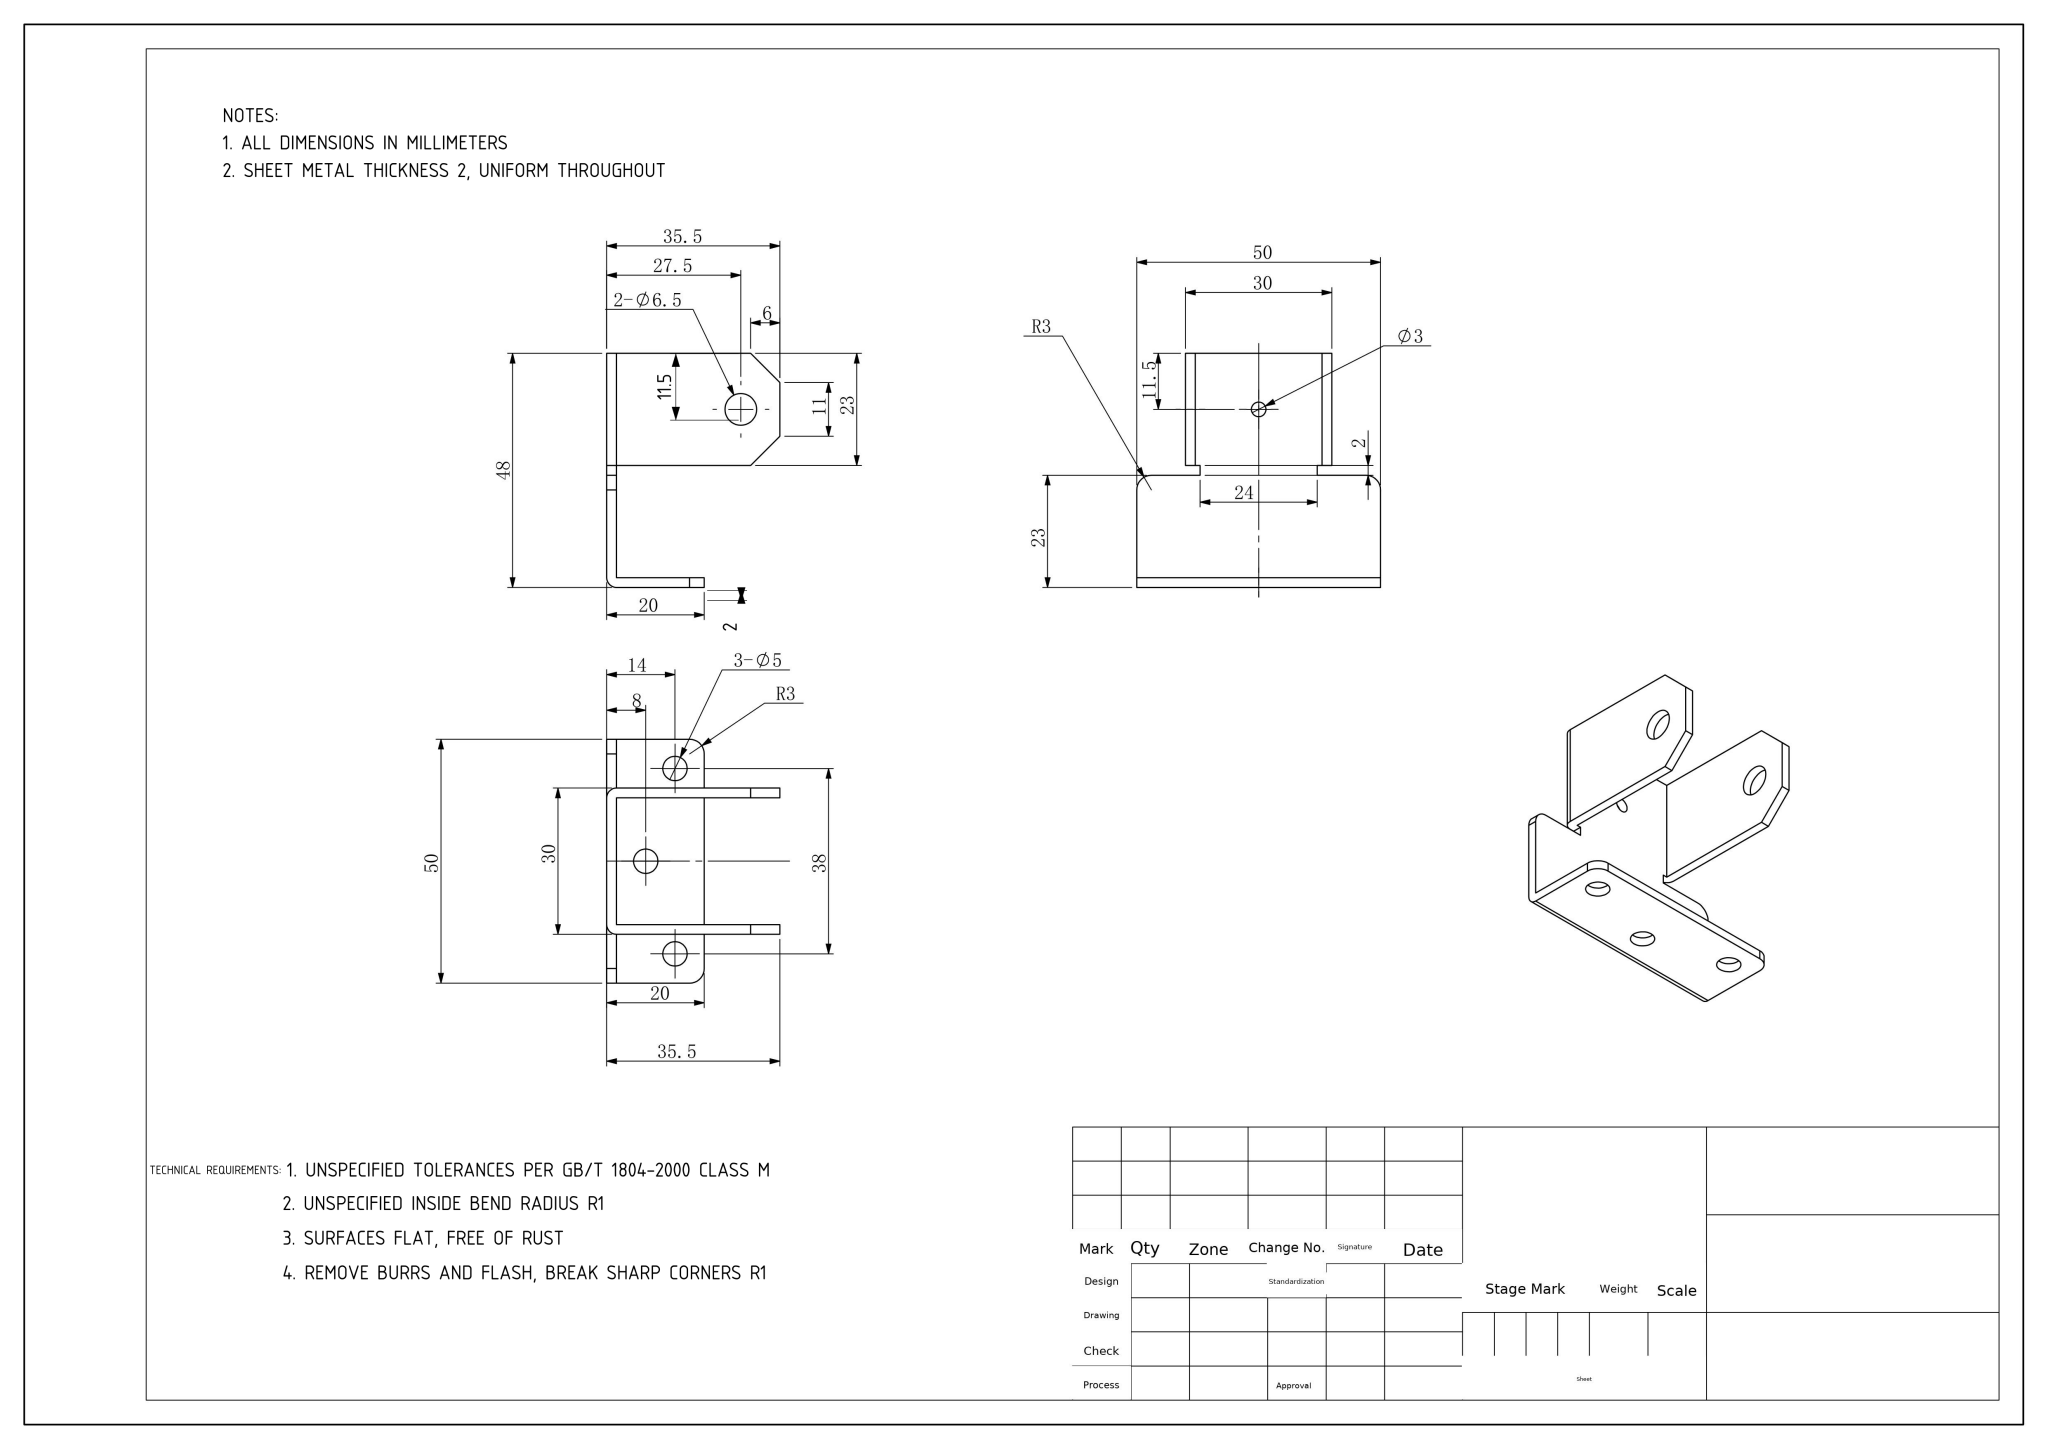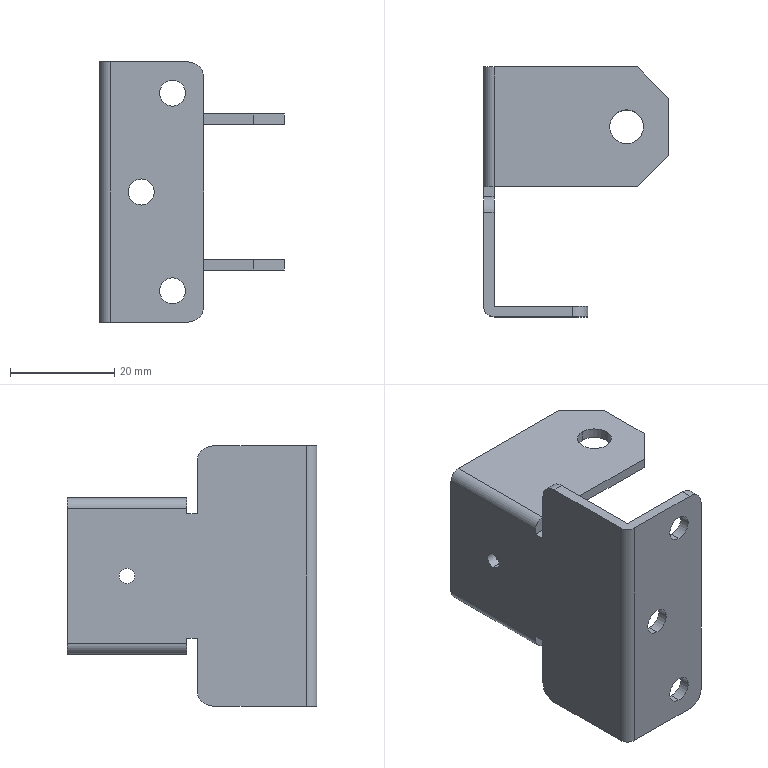Part | NX | mm | Right-Angle Twin-Arm Chamfered Mounting Bracket | 1 solid | 45 faces | box 35.5 x 48 x 50 mm | volume 8151 mm3 | plane 24 | cylinder 21 | commonest cylinder face diameters 5 x6 6.5 x4 6 x4 3 x2 4.004 x2 0.004 x2 4 x1